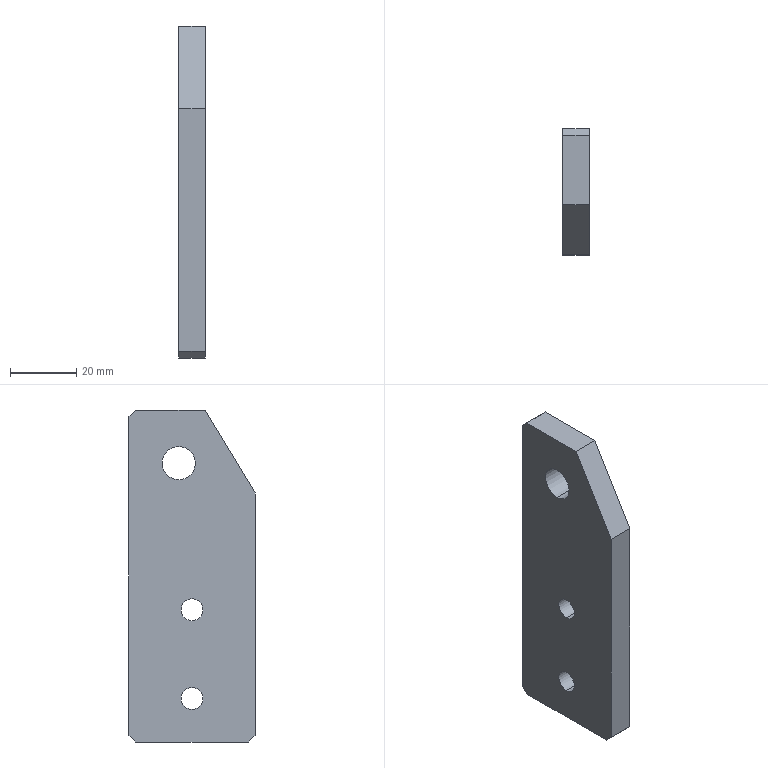Component | SolidWorks | CHEN123-AA-06-1 | 1 solid | 16 faces | box 8 x 38 x 100 mm | volume 27676 mm3 | plane 10 | cylinder 6 | commonest cylinder face diameters 6.6 x4 10 x2
build123d program:
from build123d import *

# Parameters (mm, degrees)
SKETCH1_W                  = 100
SKETCH1_H                  = 38
BOSS_EXTRUDE1_DEPTH        = 8
CUT_EXTRUDE1_DEPTH         = 55.083
CHAMFER1_SIZE              = 2
SKETCH3_R                  = 5
CUT_EXTRUDE2_DEPTH         = 55.083
F_6_6_6_6_DIAMETER_HOLE1_D = 6.6


with BuildPart() as part:
    # Sketch1 → Boss-Extrude1 (new body)
    with BuildSketch(Plane.XY):
        Rectangle(SKETCH1_W, SKETCH1_H)
    extrude(amount=BOSS_EXTRUDE1_DEPTH)

    # Sketch2 → Cut-Extrude1 (cut, through all)
    with BuildSketch(Plane.XY.offset(8)):
        Polygon((-50, -19), (-50, -4), (-25, -19), align=None)
    extrude(amount=-CUT_EXTRUDE1_DEPTH, mode=Mode.SUBTRACT)

    # Chamfer1
    chamfer1_edges = [part.edges().sort_by_distance(p)[0] for p in [
        (50, -19, 4),
        (-50, 19, 4),
        (50, 19, 4),
    ]]
    chamfer(chamfer1_edges, length=CHAMFER1_SIZE)

    # Sketch3 → Cut-Extrude2 (cut, through all)
    with BuildSketch(Plane.XY.offset(8)):
        with Locations((-34, 4)):
            Circle(SKETCH3_R)
    extrude(amount=-CUT_EXTRUDE2_DEPTH, mode=Mode.SUBTRACT)

    # 6.6 _6.6_ Diameter Hole1 (through all)
    with Locations(Plane.XY.offset(8)):
        with Locations((36.907, 0), (10.161, 0)):
            Hole(F_6_6_6_6_DIAMETER_HOLE1_D / 2)


solid = part.part

# Placed as in the assembly
solid = solid.moved(Location((20, 0.0008962, 0), (0, 90, 0)))
STEP:
#1=COLOUR_RGB('',0.7922,0.8196,0.9333);
#2=FILL_AREA_STYLE_COLOUR('',#1);
#3=FILL_AREA_STYLE('',(#2));
#4=SURFACE_STYLE_FILL_AREA(#3);
#5=SURFACE_SIDE_STYLE('',(#4));
#6=SURFACE_STYLE_USAGE(.BOTH.,#5);
#7=PRESENTATION_STYLE_ASSIGNMENT((#6));
#8=CARTESIAN_POINT('',(0.7874,0.00003528,-1.323));
#9=VERTEX_POINT('',#8);
#10=CARTESIAN_POINT('',(0.7874,0.00003528,-1.583));
#11=VERTEX_POINT('',#10);
#12=CARTESIAN_POINT('',(0.7874,0.00003528,-1.453));
#13=DIRECTION('',(1.,0.,0.));
#14=DIRECTION('',(0.,0.,-1.));
#15=AXIS2_PLACEMENT_3D('',#12,#13,#14);
#16=CIRCLE('',#15,0.1299);
#17=EDGE_CURVE('',#9,#11,#16,.T.);
#18=ORIENTED_EDGE('',*,*,#17,.F.);
#19=CARTESIAN_POINT('',(1.102,0.00003528,-1.323));
#20=VERTEX_POINT('',#19);
#21=CARTESIAN_POINT('',(1.102,0.00003528,-1.323));
#22=DIRECTION('',(1.,0.,0.));
#23=VECTOR('',#22,39.37);
#24=LINE('',#21,#23);
#25=EDGE_CURVE('',#9,#20,#24,.T.);
#26=ORIENTED_EDGE('',*,*,#25,.T.);
#27=CARTESIAN_POINT('',(1.102,0.00003528,-1.583));
#28=VERTEX_POINT('',#27);
#29=CARTESIAN_POINT('',(1.102,0.00003528,-1.453));
#30=DIRECTION('',(1.,0.,0.));
#31=DIRECTION('',(0.,0.,-1.));
#32=AXIS2_PLACEMENT_3D('',#29,#30,#31);
#33=CIRCLE('',#32,0.1299);
#34=EDGE_CURVE('',#20,#28,#33,.T.);
#35=ORIENTED_EDGE('',*,*,#34,.T.);
#36=CARTESIAN_POINT('',(1.102,0.00003528,-1.583));
#37=DIRECTION('',(1.,0.,0.));
#38=VECTOR('',#37,39.37);
#39=LINE('',#36,#38);
#40=EDGE_CURVE('',#11,#28,#39,.T.);
#41=ORIENTED_EDGE('',*,*,#40,.F.);
#42=EDGE_LOOP('',(#18,#26,#35,#41));
#43=FACE_OUTER_BOUND('',#42,.T.);
#44=CARTESIAN_POINT('',(1.102,0.00003528,-1.453));
#45=DIRECTION('',(1.,0.,0.));
#46=DIRECTION('',(0.,0.,-1.));
#47=AXIS2_PLACEMENT_3D('',#44,#45,#46);
#48=CYLINDRICAL_SURFACE('',#47,0.1299);
#49=ADVANCED_FACE('',(#43),#48,.F.);
#50=CARTESIAN_POINT('',(0.7874,0.00003528,-0.2701));
#51=VERTEX_POINT('',#50);
#52=CARTESIAN_POINT('',(0.7874,0.00003528,-0.5299));
#53=VERTEX_POINT('',#52);
#54=CARTESIAN_POINT('',(0.7874,0.00003528,-0.4));
#55=DIRECTION('',(1.,0.,0.));
#56=DIRECTION('',(0.,0.,-1.));
#57=AXIS2_PLACEMENT_3D('',#54,#55,#56);
#58=CIRCLE('',#57,0.1299);
#59=EDGE_CURVE('',#51,#53,#58,.T.);
#60=ORIENTED_EDGE('',*,*,#59,.F.);
#61=CARTESIAN_POINT('',(1.102,0.00003528,-0.2701));
#62=VERTEX_POINT('',#61);
#63=CARTESIAN_POINT('',(1.102,0.00003528,-0.2701));
#64=DIRECTION('',(1.,0.,0.));
#65=VECTOR('',#64,39.37);
#66=LINE('',#63,#65);
#67=EDGE_CURVE('',#51,#62,#66,.T.);
#68=ORIENTED_EDGE('',*,*,#67,.T.);
#69=CARTESIAN_POINT('',(1.102,0.00003528,-0.5299));
#70=VERTEX_POINT('',#69);
#71=CARTESIAN_POINT('',(1.102,0.00003528,-0.4));
#72=DIRECTION('',(1.,0.,0.));
#73=DIRECTION('',(0.,0.,-1.));
#74=AXIS2_PLACEMENT_3D('',#71,#72,#73);
#75=CIRCLE('',#74,0.1299);
#76=EDGE_CURVE('',#62,#70,#75,.T.);
#77=ORIENTED_EDGE('',*,*,#76,.T.);
#78=CARTESIAN_POINT('',(1.102,0.00003528,-0.5299));
#79=DIRECTION('',(1.,0.,0.));
#80=VECTOR('',#79,39.37);
#81=LINE('',#78,#80);
#82=EDGE_CURVE('',#53,#70,#81,.T.);
#83=ORIENTED_EDGE('',*,*,#82,.F.);
#84=EDGE_LOOP('',(#60,#68,#77,#83));
#85=FACE_OUTER_BOUND('',#84,.T.);
#86=CARTESIAN_POINT('',(1.102,0.00003528,-0.4));
#87=DIRECTION('',(1.,0.,0.));
#88=DIRECTION('',(0.,0.,-1.));
#89=AXIS2_PLACEMENT_3D('',#86,#87,#88);
#90=CYLINDRICAL_SURFACE('',#89,0.1299);
#91=ADVANCED_FACE('',(#85),#90,.F.);
#92=CARTESIAN_POINT('',(0.7874,0.1575,1.535));
#93=VERTEX_POINT('',#92);
#94=CARTESIAN_POINT('',(0.7874,0.1575,1.142));
#95=VERTEX_POINT('',#94);
#96=CARTESIAN_POINT('',(0.7874,0.1575,1.339));
#97=DIRECTION('',(1.,0.,0.));
#98=DIRECTION('',(0.,0.,-1.));
#99=AXIS2_PLACEMENT_3D('',#96,#97,#98);
#100=CIRCLE('',#99,0.1969);
#101=EDGE_CURVE('',#93,#95,#100,.T.);
#102=ORIENTED_EDGE('',*,*,#101,.F.);
#103=CARTESIAN_POINT('',(1.102,0.1575,1.535));
#104=VERTEX_POINT('',#103);
#105=CARTESIAN_POINT('',(0.7874,0.1575,1.535));
#106=DIRECTION('',(1.,0.,0.));
#107=VECTOR('',#106,39.37);
#108=LINE('',#105,#107);
#109=EDGE_CURVE('',#93,#104,#108,.T.);
#110=ORIENTED_EDGE('',*,*,#109,.T.);
#111=CARTESIAN_POINT('',(1.102,0.1575,1.142));
#112=VERTEX_POINT('',#111);
#113=CARTESIAN_POINT('',(1.102,0.1575,1.339));
#114=DIRECTION('',(1.,0.,0.));
#115=DIRECTION('',(0.,0.,-1.));
#116=AXIS2_PLACEMENT_3D('',#113,#114,#115);
#117=CIRCLE('',#116,0.1969);
#118=EDGE_CURVE('',#104,#112,#117,.T.);
#119=ORIENTED_EDGE('',*,*,#118,.T.);
#120=CARTESIAN_POINT('',(0.7874,0.1575,1.142));
#121=DIRECTION('',(1.,0.,0.));
#122=VECTOR('',#121,39.37);
#123=LINE('',#120,#122);
#124=EDGE_CURVE('',#95,#112,#123,.T.);
#125=ORIENTED_EDGE('',*,*,#124,.F.);
#126=EDGE_LOOP('',(#102,#110,#119,#125));
#127=FACE_OUTER_BOUND('',#126,.T.);
#128=CARTESIAN_POINT('',(0.7874,0.1575,1.339));
#129=DIRECTION('',(1.,0.,0.));
#130=DIRECTION('',(0.,0.,-1.));
#131=AXIS2_PLACEMENT_3D('',#128,#129,#130);
#132=CYLINDRICAL_SURFACE('',#131,0.1969);
#133=ADVANCED_FACE('',(#127),#132,.F.);
#134=CARTESIAN_POINT('',(1.102,-0.6693,-1.969));
#135=VERTEX_POINT('',#134);
#136=CARTESIAN_POINT('',(1.102,0.6693,-1.969));
#137=VERTEX_POINT('',#136);
#138=CARTESIAN_POINT('',(1.102,-0.748,-1.969));
#139=DIRECTION('',(0.,1.,0.));
#140=VECTOR('',#139,39.37);
#141=LINE('',#138,#140);
#142=EDGE_CURVE('',#135,#137,#141,.T.);
#143=ORIENTED_EDGE('',*,*,#142,.F.);
#144=CARTESIAN_POINT('',(0.7874,-0.6693,-1.969));
#145=VERTEX_POINT('',#144);
#146=CARTESIAN_POINT('',(1.102,-0.6693,-1.969));
#147=DIRECTION('',(-1.,0.,0.));
#148=VECTOR('',#147,39.37);
#149=LINE('',#146,#148);
#150=EDGE_CURVE('',#135,#145,#149,.T.);
#151=ORIENTED_EDGE('',*,*,#150,.T.);
#152=CARTESIAN_POINT('',(0.7874,0.6693,-1.969));
#153=VERTEX_POINT('',#152);
#154=CARTESIAN_POINT('',(0.7874,-0.748,-1.969));
#155=DIRECTION('',(0.,1.,0.));
#156=VECTOR('',#155,39.37);
#157=LINE('',#154,#156);
#158=EDGE_CURVE('',#145,#153,#157,.T.);
#159=ORIENTED_EDGE('',*,*,#158,.T.);
#160=CARTESIAN_POINT('',(1.102,0.6693,-1.969));
#161=DIRECTION('',(1.,0.,0.));
#162=VECTOR('',#161,39.37);
#163=LINE('',#160,#162);
#164=EDGE_CURVE('',#153,#137,#163,.T.);
#165=ORIENTED_EDGE('',*,*,#164,.T.);
#166=EDGE_LOOP('',(#143,#151,#159,#165));
#167=FACE_OUTER_BOUND('',#166,.T.);
#168=CARTESIAN_POINT('',(1.102,-0.748,-1.969));
#169=DIRECTION('',(0.,0.,1.));
#170=DIRECTION('',(1.,0.,0.));
#171=AXIS2_PLACEMENT_3D('',#168,#169,#170);
#172=PLANE('',#171);
#173=ADVANCED_FACE('',(#167),#172,.F.);
#174=CARTESIAN_POINT('',(1.102,0.7481,-1.89));
#175=VERTEX_POINT('',#174);
#176=CARTESIAN_POINT('',(1.102,0.7481,1.89));
#177=VERTEX_POINT('',#176);
#178=CARTESIAN_POINT('',(1.102,0.7481,1.969));
#179=DIRECTION('',(0.,0.,1.));
#180=VECTOR('',#179,39.37);
#181=LINE('',#178,#180);
#182=EDGE_CURVE('',#175,#177,#181,.T.);
#183=ORIENTED_EDGE('',*,*,#182,.F.);
#184=CARTESIAN_POINT('',(0.7874,0.7481,-1.89));
#185=VERTEX_POINT('',#184);
#186=CARTESIAN_POINT('',(1.102,0.7481,-1.89));
#187=DIRECTION('',(-1.,0.,0.));
#188=VECTOR('',#187,39.37);
#189=LINE('',#186,#188);
#190=EDGE_CURVE('',#175,#185,#189,.T.);
#191=ORIENTED_EDGE('',*,*,#190,.T.);
#192=CARTESIAN_POINT('',(0.7874,0.7481,1.89));
#193=VERTEX_POINT('',#192);
#194=CARTESIAN_POINT('',(0.7874,0.7481,1.969));
#195=DIRECTION('',(0.,0.,1.));
#196=VECTOR('',#195,39.37);
#197=LINE('',#194,#196);
#198=EDGE_CURVE('',#185,#193,#197,.T.);
#199=ORIENTED_EDGE('',*,*,#198,.T.);
#200=CARTESIAN_POINT('',(1.102,0.7481,1.89));
#201=DIRECTION('',(1.,0.,0.));
#202=VECTOR('',#201,39.37);
#203=LINE('',#200,#202);
#204=EDGE_CURVE('',#193,#177,#203,.T.);
#205=ORIENTED_EDGE('',*,*,#204,.T.);
#206=EDGE_LOOP('',(#183,#191,#199,#205));
#207=FACE_OUTER_BOUND('',#206,.T.);
#208=CARTESIAN_POINT('',(1.102,0.7481,1.969));
#209=DIRECTION('',(0.,-1.,0.));
#210=DIRECTION('',(-1.,0.,0.));
#211=AXIS2_PLACEMENT_3D('',#208,#209,#210);
#212=PLANE('',#211);
#213=ADVANCED_FACE('',(#207),#212,.F.);
#214=CARTESIAN_POINT('',(1.102,0.6693,1.969));
#215=VERTEX_POINT('',#214);
#216=CARTESIAN_POINT('',(1.102,-0.1574,1.969));
#217=VERTEX_POINT('',#216);
#218=CARTESIAN_POINT('',(1.102,-0.748,1.969));
#219=DIRECTION('',(0.,-1.,0.));
#220=VECTOR('',#219,39.37);
#221=LINE('',#218,#220);
#222=EDGE_CURVE('',#215,#217,#221,.T.);
#223=ORIENTED_EDGE('',*,*,#222,.F.);
#224=CARTESIAN_POINT('',(0.7874,0.6693,1.969));
#225=VERTEX_POINT('',#224);
#226=CARTESIAN_POINT('',(1.102,0.6693,1.969));
#227=DIRECTION('',(-1.,0.,0.));
#228=VECTOR('',#227,39.37);
#229=LINE('',#226,#228);
#230=EDGE_CURVE('',#215,#225,#229,.T.);
#231=ORIENTED_EDGE('',*,*,#230,.T.);
#232=CARTESIAN_POINT('',(0.7874,-0.1574,1.969));
#233=VERTEX_POINT('',#232);
#234=CARTESIAN_POINT('',(0.7874,-0.748,1.969));
#235=DIRECTION('',(0.,-1.,0.));
#236=VECTOR('',#235,39.37);
#237=LINE('',#234,#236);
#238=EDGE_CURVE('',#225,#233,#237,.T.);
#239=ORIENTED_EDGE('',*,*,#238,.T.);
#240=CARTESIAN_POINT('',(0.7874,-0.1574,1.969));
#241=DIRECTION('',(1.,0.,0.));
#242=VECTOR('',#241,39.37);
#243=LINE('',#240,#242);
#244=EDGE_CURVE('',#233,#217,#243,.T.);
#245=ORIENTED_EDGE('',*,*,#244,.T.);
#246=EDGE_LOOP('',(#223,#231,#239,#245));
#247=FACE_OUTER_BOUND('',#246,.T.);
#248=CARTESIAN_POINT('',(1.102,-0.748,1.969));
#249=DIRECTION('',(0.,0.,-1.));
#250=DIRECTION('',(-1.,0.,0.));
#251=AXIS2_PLACEMENT_3D('',#248,#249,#250);
#252=PLANE('',#251);
#253=ADVANCED_FACE('',(#247),#252,.F.);
#254=CARTESIAN_POINT('',(0.7874,-0.748,0.9843));
#255=VERTEX_POINT('',#254);
#256=CARTESIAN_POINT('',(0.7874,-0.748,-1.89));
#257=VERTEX_POINT('',#256);
#258=CARTESIAN_POINT('',(0.7874,-0.748,1.969));
#259=DIRECTION('',(0.,0.,-1.));
#260=VECTOR('',#259,39.37);
#261=LINE('',#258,#260);
#262=EDGE_CURVE('',#255,#257,#261,.T.);
#263=ORIENTED_EDGE('',*,*,#262,.T.);
#264=CARTESIAN_POINT('',(1.102,-0.748,-1.89));
#265=VERTEX_POINT('',#264);
#266=CARTESIAN_POINT('',(1.102,-0.748,-1.89));
#267=DIRECTION('',(1.,0.,0.));
#268=VECTOR('',#267,39.37);
#269=LINE('',#266,#268);
#270=EDGE_CURVE('',#257,#265,#269,.T.);
#271=ORIENTED_EDGE('',*,*,#270,.T.);
#272=CARTESIAN_POINT('',(1.102,-0.748,0.9843));
#273=VERTEX_POINT('',#272);
#274=CARTESIAN_POINT('',(1.102,-0.748,1.969));
#275=DIRECTION('',(0.,0.,-1.));
#276=VECTOR('',#275,39.37);
#277=LINE('',#274,#276);
#278=EDGE_CURVE('',#273,#265,#277,.T.);
#279=ORIENTED_EDGE('',*,*,#278,.F.);
#280=CARTESIAN_POINT('',(0.7874,-0.748,0.9843));
#281=DIRECTION('',(1.,0.,0.));
#282=VECTOR('',#281,39.37);
#283=LINE('',#280,#282);
#284=EDGE_CURVE('',#255,#273,#283,.T.);
#285=ORIENTED_EDGE('',*,*,#284,.F.);
#286=EDGE_LOOP('',(#263,#271,#279,#285));
#287=FACE_OUTER_BOUND('',#286,.T.);
#288=CARTESIAN_POINT('',(1.102,-0.748,1.969));
#289=DIRECTION('',(0.,1.,0.));
#290=DIRECTION('',(1.,0.,0.));
#291=AXIS2_PLACEMENT_3D('',#288,#289,#290);
#292=PLANE('',#291);
#293=ADVANCED_FACE('',(#287),#292,.F.);
#294=CARTESIAN_POINT('',(1.102,0.00003528,-1.453));
#295=DIRECTION('',(1.,0.,0.));
#296=DIRECTION('',(0.,0.,-1.));
#297=AXIS2_PLACEMENT_3D('',#294,#295,#296);
#298=CIRCLE('',#297,0.1299);
#299=EDGE_CURVE('',#28,#20,#298,.T.);
#300=ORIENTED_EDGE('',*,*,#299,.F.);
#301=ORIENTED_EDGE('',*,*,#34,.F.);
#302=EDGE_LOOP('',(#300,#301));
#303=FACE_BOUND('',#302,.T.);
#304=CARTESIAN_POINT('',(1.102,0.00003528,-0.4));
#305=DIRECTION('',(1.,0.,0.));
#306=DIRECTION('',(0.,0.,-1.));
#307=AXIS2_PLACEMENT_3D('',#304,#305,#306);
#308=CIRCLE('',#307,0.1299);
#309=EDGE_CURVE('',#70,#62,#308,.T.);
#310=ORIENTED_EDGE('',*,*,#309,.F.);
#311=ORIENTED_EDGE('',*,*,#76,.F.);
#312=EDGE_LOOP('',(#310,#311));
#313=FACE_BOUND('',#312,.T.);
#314=CARTESIAN_POINT('',(1.102,0.1575,1.339));
#315=DIRECTION('',(1.,0.,0.));
#316=DIRECTION('',(0.,0.,-1.));
#317=AXIS2_PLACEMENT_3D('',#314,#315,#316);
#318=CIRCLE('',#317,0.1969);
#319=EDGE_CURVE('',#112,#104,#318,.T.);
#320=ORIENTED_EDGE('',*,*,#319,.F.);
#321=ORIENTED_EDGE('',*,*,#118,.F.);
#322=EDGE_LOOP('',(#320,#321));
#323=FACE_BOUND('',#322,.T.);
#324=ORIENTED_EDGE('',*,*,#278,.T.);
#325=CARTESIAN_POINT('',(1.102,-0.6693,-1.969));
#326=DIRECTION('',(0.,0.7071,-0.7071));
#327=VECTOR('',#326,39.37);
#328=LINE('',#325,#327);
#329=EDGE_CURVE('',#265,#135,#328,.T.);
#330=ORIENTED_EDGE('',*,*,#329,.T.);
#331=ORIENTED_EDGE('',*,*,#142,.T.);
#332=CARTESIAN_POINT('',(1.102,0.7481,-1.89));
#333=DIRECTION('',(0.,0.7071,0.7071));
#334=VECTOR('',#333,39.37);
#335=LINE('',#332,#334);
#336=EDGE_CURVE('',#137,#175,#335,.T.);
#337=ORIENTED_EDGE('',*,*,#336,.T.);
#338=ORIENTED_EDGE('',*,*,#182,.T.);
#339=CARTESIAN_POINT('',(1.102,0.6693,1.969));
#340=DIRECTION('',(0.,-0.7071,0.7071));
#341=VECTOR('',#340,39.37);
#342=LINE('',#339,#341);
#343=EDGE_CURVE('',#177,#215,#342,.T.);
#344=ORIENTED_EDGE('',*,*,#343,.T.);
#345=ORIENTED_EDGE('',*,*,#222,.T.);
#346=CARTESIAN_POINT('',(1.102,-0.1574,1.969));
#347=DIRECTION('',(0.,0.5145,0.8575));
#348=VECTOR('',#347,39.37);
#349=LINE('',#346,#348);
#350=EDGE_CURVE('',#273,#217,#349,.T.);
#351=ORIENTED_EDGE('',*,*,#350,.F.);
#352=EDGE_LOOP('',(#324,#330,#331,#337,#338,#344,#345,#351));
#353=FACE_OUTER_BOUND('',#352,.T.);
#354=CARTESIAN_POINT('',(1.102,0.00003528,0.));
#355=DIRECTION('',(-1.,0.,0.));
#356=DIRECTION('',(0.,0.,1.));
#357=AXIS2_PLACEMENT_3D('',#354,#355,#356);
#358=PLANE('',#357);
#359=ADVANCED_FACE('',(#303,#313,#323,#353),#358,.F.);
#360=CARTESIAN_POINT('',(0.7874,0.00003528,-1.453));
#361=DIRECTION('',(1.,0.,0.));
#362=DIRECTION('',(0.,0.,-1.));
#363=AXIS2_PLACEMENT_3D('',#360,#361,#362);
#364=CIRCLE('',#363,0.1299);
#365=EDGE_CURVE('',#11,#9,#364,.T.);
#366=ORIENTED_EDGE('',*,*,#365,.T.);
#367=ORIENTED_EDGE('',*,*,#17,.T.);
#368=EDGE_LOOP('',(#366,#367));
#369=FACE_BOUND('',#368,.T.);
#370=CARTESIAN_POINT('',(0.7874,0.00003528,-0.4));
#371=DIRECTION('',(1.,0.,0.));
#372=DIRECTION('',(0.,0.,-1.));
#373=AXIS2_PLACEMENT_3D('',#370,#371,#372);
#374=CIRCLE('',#373,0.1299);
#375=EDGE_CURVE('',#53,#51,#374,.T.);
#376=ORIENTED_EDGE('',*,*,#375,.T.);
#377=ORIENTED_EDGE('',*,*,#59,.T.);
#378=EDGE_LOOP('',(#376,#377));
#379=FACE_BOUND('',#378,.T.);
#380=CARTESIAN_POINT('',(0.7874,0.1575,1.339));
#381=DIRECTION('',(1.,0.,0.));
#382=DIRECTION('',(0.,0.,-1.));
#383=AXIS2_PLACEMENT_3D('',#380,#381,#382);
#384=CIRCLE('',#383,0.1969);
#385=EDGE_CURVE('',#95,#93,#384,.T.);
#386=ORIENTED_EDGE('',*,*,#385,.T.);
#387=ORIENTED_EDGE('',*,*,#101,.T.);
#388=EDGE_LOOP('',(#386,#387));
#389=FACE_BOUND('',#388,.T.);
#390=ORIENTED_EDGE('',*,*,#158,.F.);
#391=CARTESIAN_POINT('',(0.7874,-1.319,-1.319));
#392=DIRECTION('',(0.,-0.7071,0.7071));
#393=VECTOR('',#392,39.37);
#394=LINE('',#391,#393);
#395=EDGE_CURVE('',#145,#257,#394,.T.);
#396=ORIENTED_EDGE('',*,*,#395,.T.);
#397=ORIENTED_EDGE('',*,*,#262,.F.);
#398=CARTESIAN_POINT('',(0.7874,-0.1574,1.969));
#399=DIRECTION('',(0.,0.5145,0.8575));
#400=VECTOR('',#399,39.37);
#401=LINE('',#398,#400);
#402=EDGE_CURVE('',#255,#233,#401,.T.);
#403=ORIENTED_EDGE('',*,*,#402,.T.);
#404=ORIENTED_EDGE('',*,*,#238,.F.);
#405=CARTESIAN_POINT('',(0.7874,1.319,1.319));
#406=DIRECTION('',(0.,0.7071,-0.7071));
#407=VECTOR('',#406,39.37);
#408=LINE('',#405,#407);
#409=EDGE_CURVE('',#225,#193,#408,.T.);
#410=ORIENTED_EDGE('',*,*,#409,.T.);
#411=ORIENTED_EDGE('',*,*,#198,.F.);
#412=CARTESIAN_POINT('',(0.7874,1.319,-1.319));
#413=DIRECTION('',(0.,-0.7071,-0.7071));
#414=VECTOR('',#413,39.37);
#415=LINE('',#412,#414);
#416=EDGE_CURVE('',#185,#153,#415,.T.);
#417=ORIENTED_EDGE('',*,*,#416,.T.);
#418=EDGE_LOOP('',(#390,#396,#397,#403,#404,#410,#411,#417));
#419=FACE_OUTER_BOUND('',#418,.T.);
#420=CARTESIAN_POINT('',(0.7874,0.00003528,0.));
#421=DIRECTION('',(-1.,0.,0.));
#422=DIRECTION('',(0.,0.,1.));
#423=AXIS2_PLACEMENT_3D('',#420,#421,#422);
#424=PLANE('',#423);
#425=ADVANCED_FACE('',(#369,#379,#389,#419),#424,.T.);
#426=ORIENTED_EDGE('',*,*,#350,.T.);
#427=ORIENTED_EDGE('',*,*,#244,.F.);
#428=ORIENTED_EDGE('',*,*,#402,.F.);
#429=ORIENTED_EDGE('',*,*,#284,.T.);
#430=EDGE_LOOP('',(#426,#427,#428,#429));
#431=FACE_OUTER_BOUND('',#430,.T.);
#432=CARTESIAN_POINT('',(0.7874,-0.1574,1.969));
#433=DIRECTION('',(0.,0.8575,-0.5145));
#434=DIRECTION('',(0.,0.5145,0.8575));
#435=AXIS2_PLACEMENT_3D('',#432,#433,#434);
#436=PLANE('',#435);
#437=ADVANCED_FACE('',(#431),#436,.F.);
#438=ORIENTED_EDGE('',*,*,#329,.F.);
#439=ORIENTED_EDGE('',*,*,#270,.F.);
#440=ORIENTED_EDGE('',*,*,#395,.F.);
#441=ORIENTED_EDGE('',*,*,#150,.F.);
#442=EDGE_LOOP('',(#438,#439,#440,#441));
#443=FACE_OUTER_BOUND('',#442,.T.);
#444=CARTESIAN_POINT('',(1.102,-0.6693,-1.969));
#445=DIRECTION('',(0.,0.7071,0.7071));
#446=DIRECTION('',(-1.,0.,0.));
#447=AXIS2_PLACEMENT_3D('',#444,#445,#446);
#448=PLANE('',#447);
#449=ADVANCED_FACE('',(#443),#448,.F.);
#450=ORIENTED_EDGE('',*,*,#336,.F.);
#451=ORIENTED_EDGE('',*,*,#164,.F.);
#452=ORIENTED_EDGE('',*,*,#416,.F.);
#453=ORIENTED_EDGE('',*,*,#190,.F.);
#454=EDGE_LOOP('',(#450,#451,#452,#453));
#455=FACE_OUTER_BOUND('',#454,.T.);
#456=CARTESIAN_POINT('',(1.102,0.7481,-1.89));
#457=DIRECTION('',(0.,-0.7071,0.7071));
#458=DIRECTION('',(-1.,0.,0.));
#459=AXIS2_PLACEMENT_3D('',#456,#457,#458);
#460=PLANE('',#459);
#461=ADVANCED_FACE('',(#455),#460,.F.);
#462=ORIENTED_EDGE('',*,*,#343,.F.);
#463=ORIENTED_EDGE('',*,*,#204,.F.);
#464=ORIENTED_EDGE('',*,*,#409,.F.);
#465=ORIENTED_EDGE('',*,*,#230,.F.);
#466=EDGE_LOOP('',(#462,#463,#464,#465));
#467=FACE_OUTER_BOUND('',#466,.T.);
#468=CARTESIAN_POINT('',(1.102,0.6693,1.969));
#469=DIRECTION('',(0.,-0.7071,-0.7071));
#470=DIRECTION('',(-1.,0.,0.));
#471=AXIS2_PLACEMENT_3D('',#468,#469,#470);
#472=PLANE('',#471);
#473=ADVANCED_FACE('',(#467),#472,.F.);
#474=ORIENTED_EDGE('',*,*,#109,.F.);
#475=ORIENTED_EDGE('',*,*,#385,.F.);
#476=ORIENTED_EDGE('',*,*,#124,.T.);
#477=ORIENTED_EDGE('',*,*,#319,.T.);
#478=EDGE_LOOP('',(#474,#475,#476,#477));
#479=FACE_OUTER_BOUND('',#478,.T.);
#480=CARTESIAN_POINT('',(0.7874,0.1575,1.339));
#481=DIRECTION('',(1.,0.,0.));
#482=DIRECTION('',(0.,0.,-1.));
#483=AXIS2_PLACEMENT_3D('',#480,#481,#482);
#484=CYLINDRICAL_SURFACE('',#483,0.1969);
#485=ADVANCED_FACE('',(#479),#484,.F.);
#486=ORIENTED_EDGE('',*,*,#67,.F.);
#487=ORIENTED_EDGE('',*,*,#375,.F.);
#488=ORIENTED_EDGE('',*,*,#82,.T.);
#489=ORIENTED_EDGE('',*,*,#309,.T.);
#490=EDGE_LOOP('',(#486,#487,#488,#489));
#491=FACE_OUTER_BOUND('',#490,.T.);
#492=CARTESIAN_POINT('',(1.102,0.00003528,-0.4));
#493=DIRECTION('',(1.,0.,0.));
#494=DIRECTION('',(0.,0.,-1.));
#495=AXIS2_PLACEMENT_3D('',#492,#493,#494);
#496=CYLINDRICAL_SURFACE('',#495,0.1299);
#497=ADVANCED_FACE('',(#491),#496,.F.);
#498=ORIENTED_EDGE('',*,*,#25,.F.);
#499=ORIENTED_EDGE('',*,*,#365,.F.);
#500=ORIENTED_EDGE('',*,*,#40,.T.);
#501=ORIENTED_EDGE('',*,*,#299,.T.);
#502=EDGE_LOOP('',(#498,#499,#500,#501));
#503=FACE_OUTER_BOUND('',#502,.T.);
#504=CARTESIAN_POINT('',(1.102,0.00003528,-1.453));
#505=DIRECTION('',(1.,0.,0.));
#506=DIRECTION('',(0.,0.,-1.));
#507=AXIS2_PLACEMENT_3D('',#504,#505,#506);
#508=CYLINDRICAL_SURFACE('',#507,0.1299);
#509=ADVANCED_FACE('',(#503),#508,.F.);
#510=CLOSED_SHELL('',(#49,#91,#133,#173,#213,#253,#293,#359,#425,#437,#449,#461,#473,#485,#497,#509));
#511=MANIFOLD_SOLID_BREP('',#510);
#512=STYLED_ITEM('',(#7),#511);
#513=PRESENTATION_LAYER_ASSIGNMENT('','',(#512));
#514=CARTESIAN_POINT('',(0.,0.,0.));
#515=DIRECTION('',(0.,0.,1.));
#516=DIRECTION('',(1.,0.,0.));
#517=AXIS2_PLACEMENT_3D('',#514,#515,#516);
#518=(LENGTH_UNIT()NAMED_UNIT(*)SI_UNIT($,.METRE.));
#519=LENGTH_MEASURE_WITH_UNIT(LENGTH_MEASURE(0.0254),#518);
#520=DIMENSIONAL_EXPONENTS(1.,0.,0.,0.,0.,0.,0.);
#521=(CONVERSION_BASED_UNIT('',#519)LENGTH_UNIT()NAMED_UNIT(#520));
#522=UNCERTAINTY_MEASURE_WITH_UNIT(LENGTH_MEASURE(0.00001),#521,'','');
#523=(NAMED_UNIT(*)PLANE_ANGLE_UNIT()SI_UNIT($,.RADIAN.));
#524=(NAMED_UNIT(*)SI_UNIT($,.STERADIAN.)SOLID_ANGLE_UNIT());
#525=(GEOMETRIC_REPRESENTATION_CONTEXT(3)GLOBAL_UNCERTAINTY_ASSIGNED_CONTEXT((#522))GLOBAL_UNIT_ASSIGNED_CONTEXT((#521,#523,#524))REPRESENTATION_CONTEXT('',''));
#526=ADVANCED_BREP_SHAPE_REPRESENTATION('',(#511,#517),#525);
#527=(LENGTH_UNIT()NAMED_UNIT(*)SI_UNIT($,.METRE.));
#528=LENGTH_MEASURE_WITH_UNIT(LENGTH_MEASURE(0.0254),#527);
#529=DIMENSIONAL_EXPONENTS(1.,0.,0.,0.,0.,0.,0.);
#530=(CONVERSION_BASED_UNIT('',#528)LENGTH_UNIT()NAMED_UNIT(#529));
#531=UNCERTAINTY_MEASURE_WITH_UNIT(LENGTH_MEASURE(0.00001),#530,'','');
#532=(NAMED_UNIT(*)PLANE_ANGLE_UNIT()SI_UNIT($,.RADIAN.));
#533=(NAMED_UNIT(*)SI_UNIT($,.STERADIAN.)SOLID_ANGLE_UNIT());
#534=(GEOMETRIC_REPRESENTATION_CONTEXT(3)GLOBAL_UNCERTAINTY_ASSIGNED_CONTEXT((#531))GLOBAL_UNIT_ASSIGNED_CONTEXT((#530,#532,#533))REPRESENTATION_CONTEXT('',''));
#535=MECHANICAL_DESIGN_GEOMETRIC_PRESENTATION_REPRESENTATION('',(#512),#534);